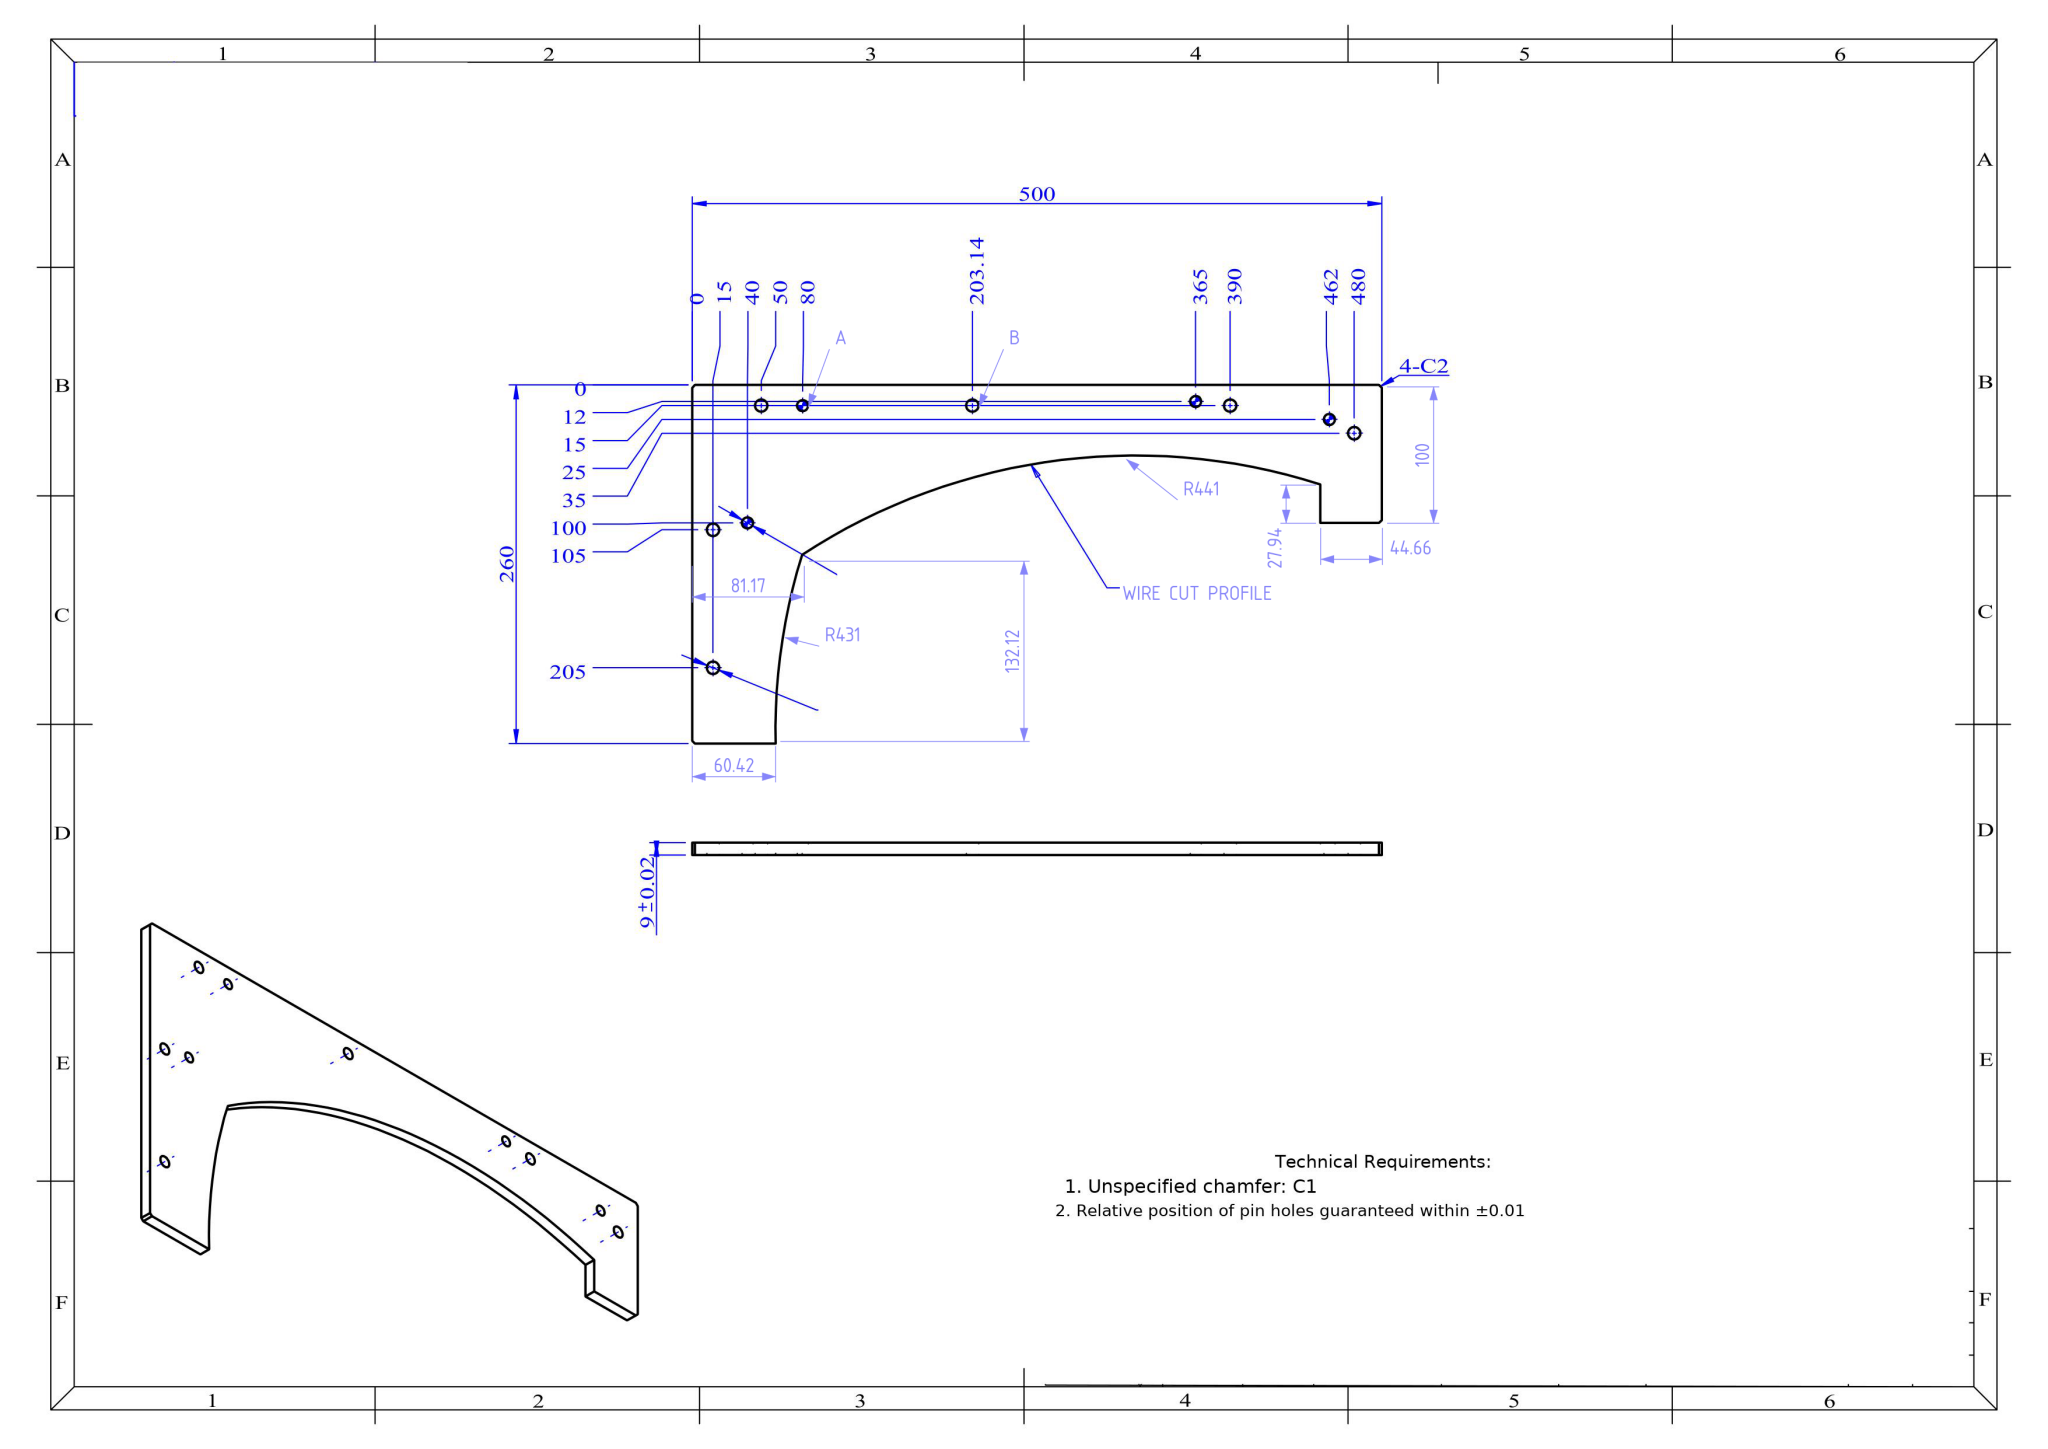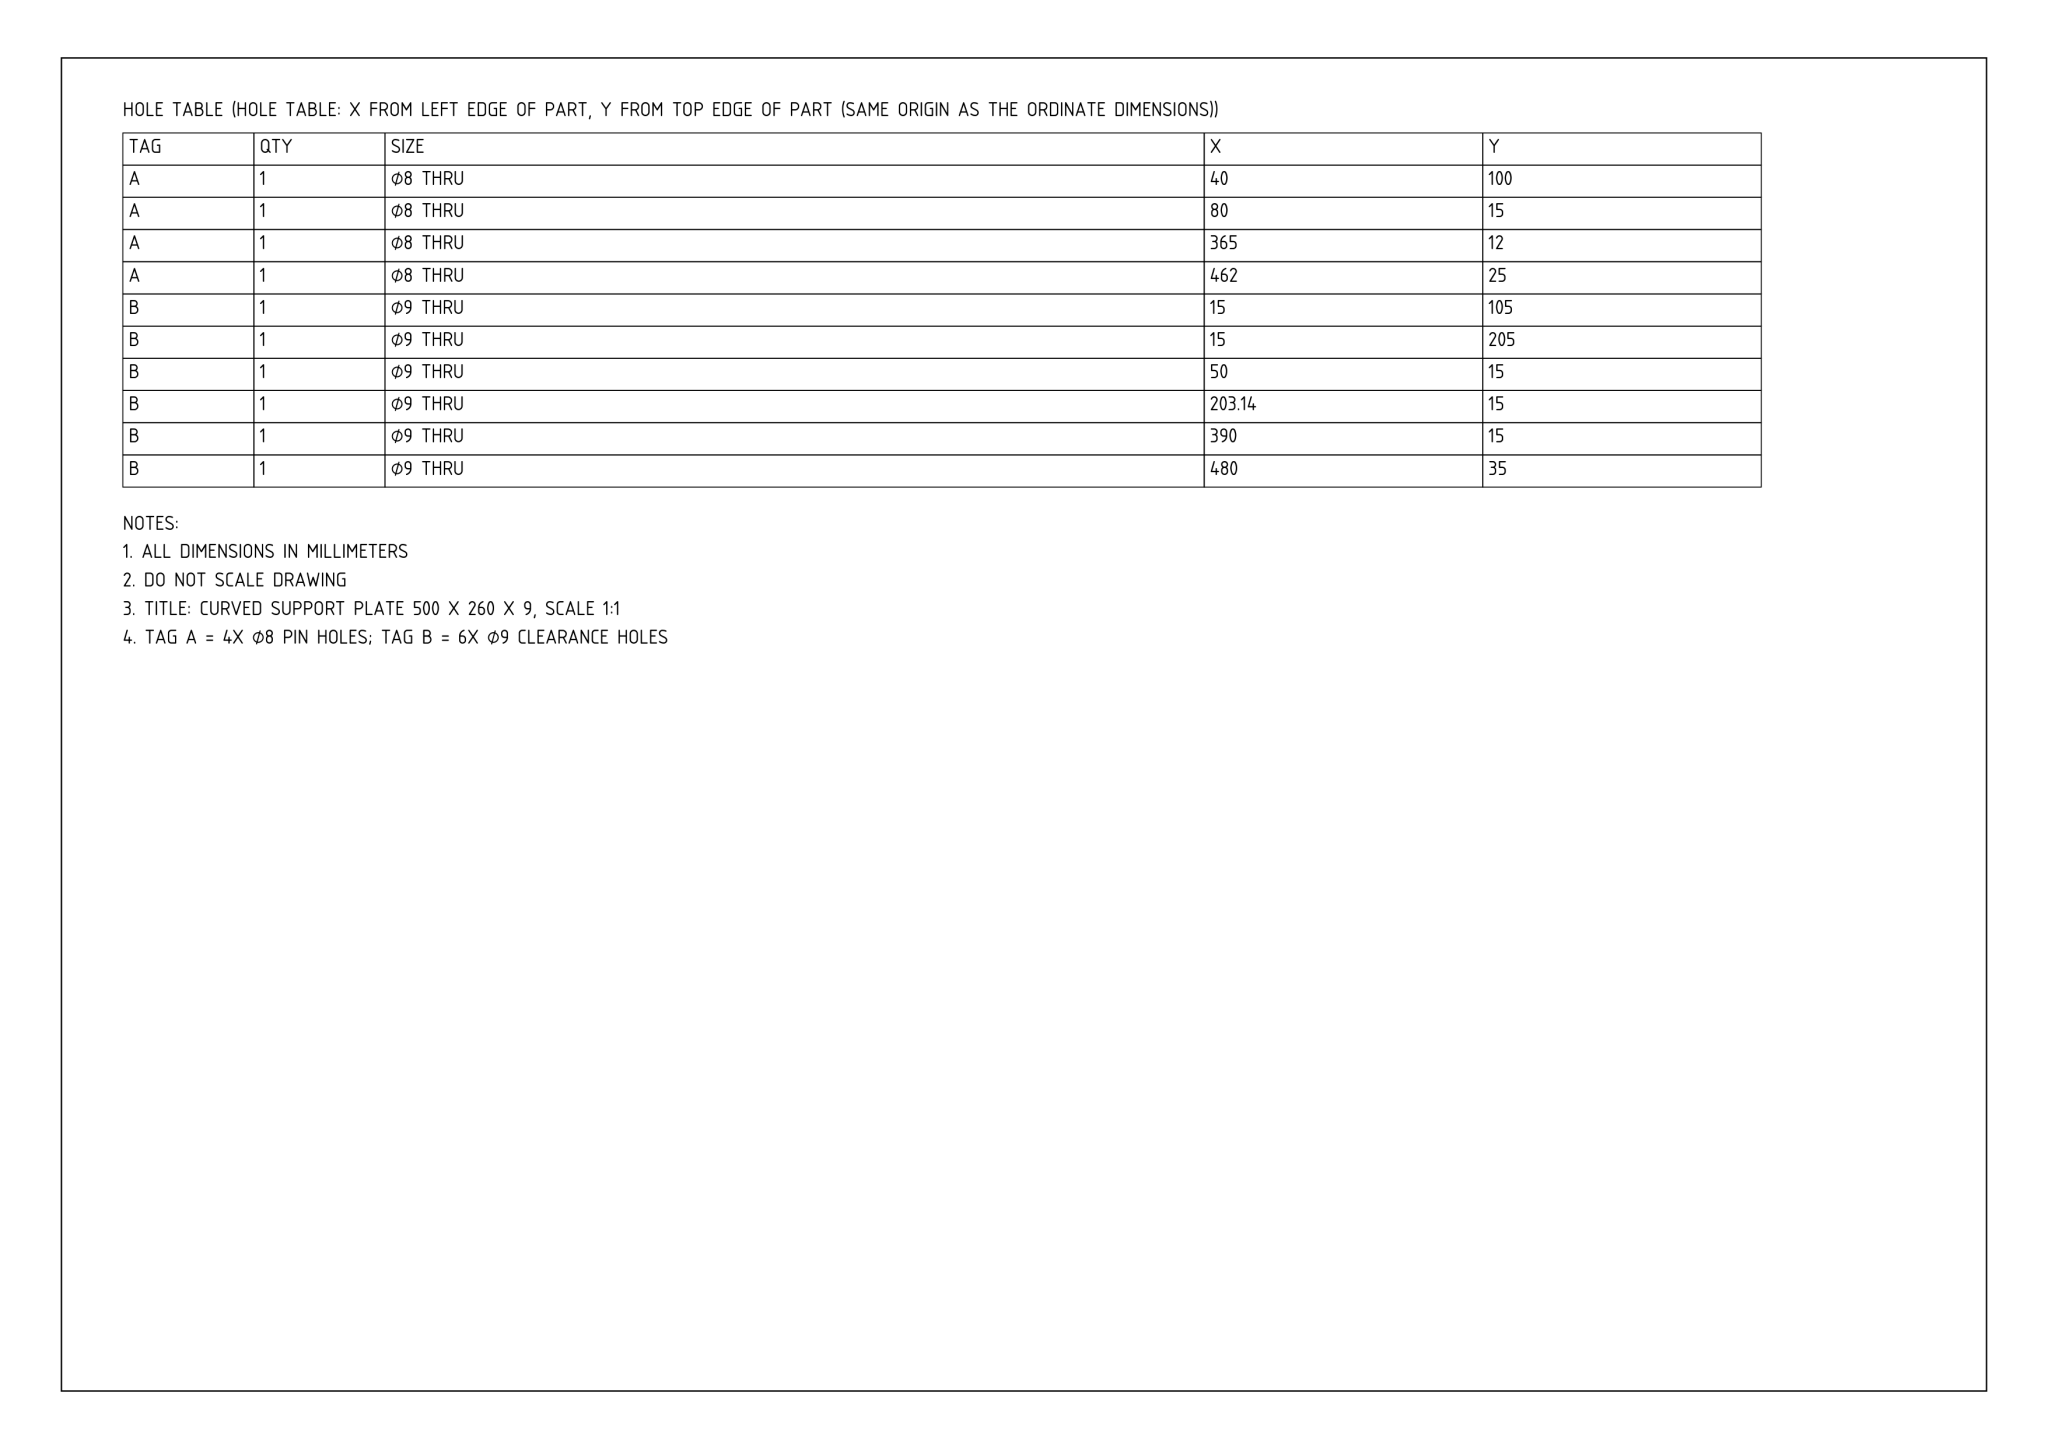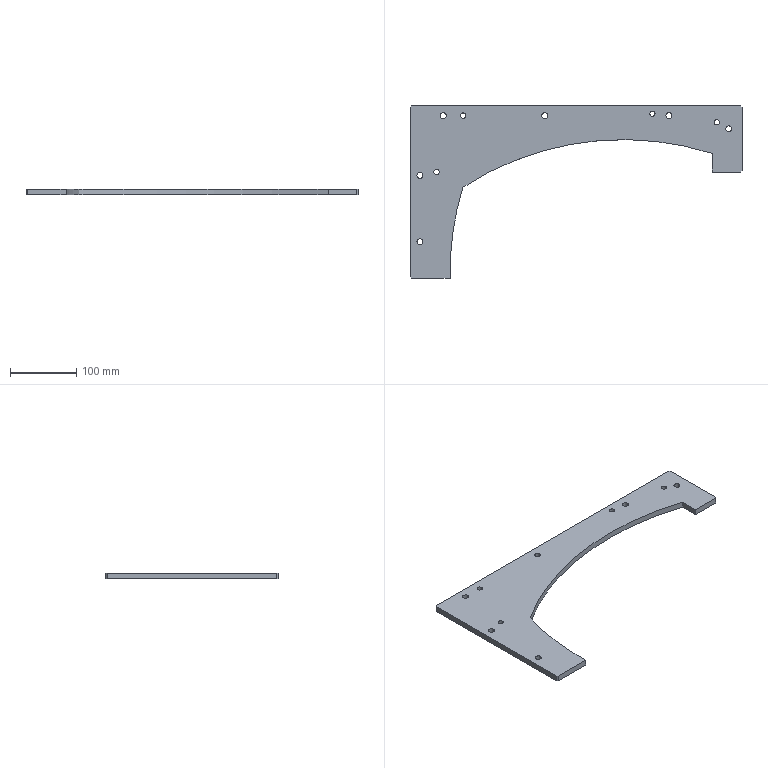Part | NX | mm | 1 solid | 34 faces | box 500 x 260 x 9 mm | volume 436370 mm3 | cylinder 22 | plane 12 | commonest cylinder face diameters 9 x12 8 x8 882 x1 862 x1